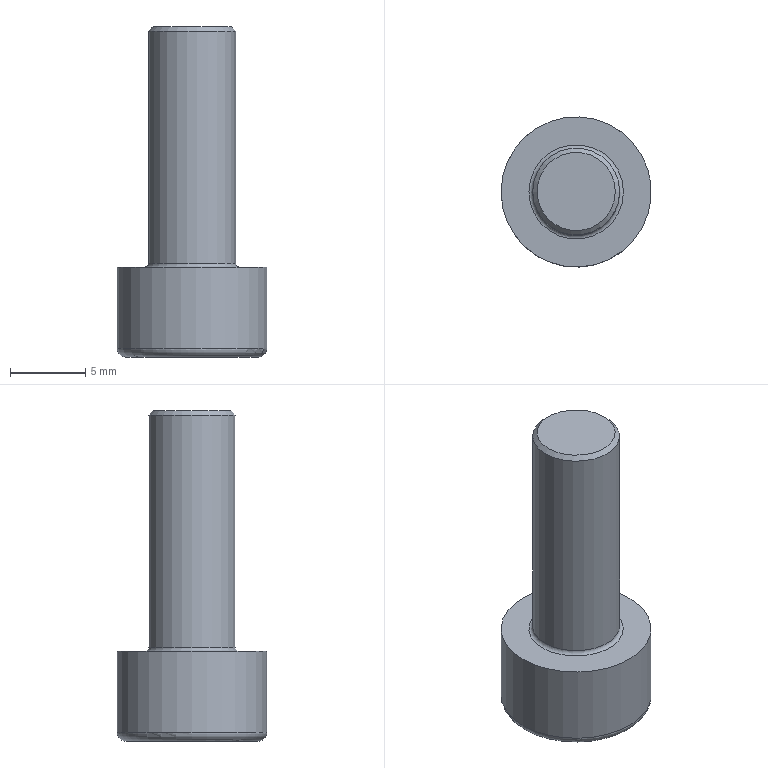Component | NX | GB-T70_1-2000_M6X16 | 1 solid | 27 faces | volume 800 mm3 | plane 15 | cone 8 | cylinder 2 | torus 2 | commonest cylinder face diameters 5.795 x1 10 x1